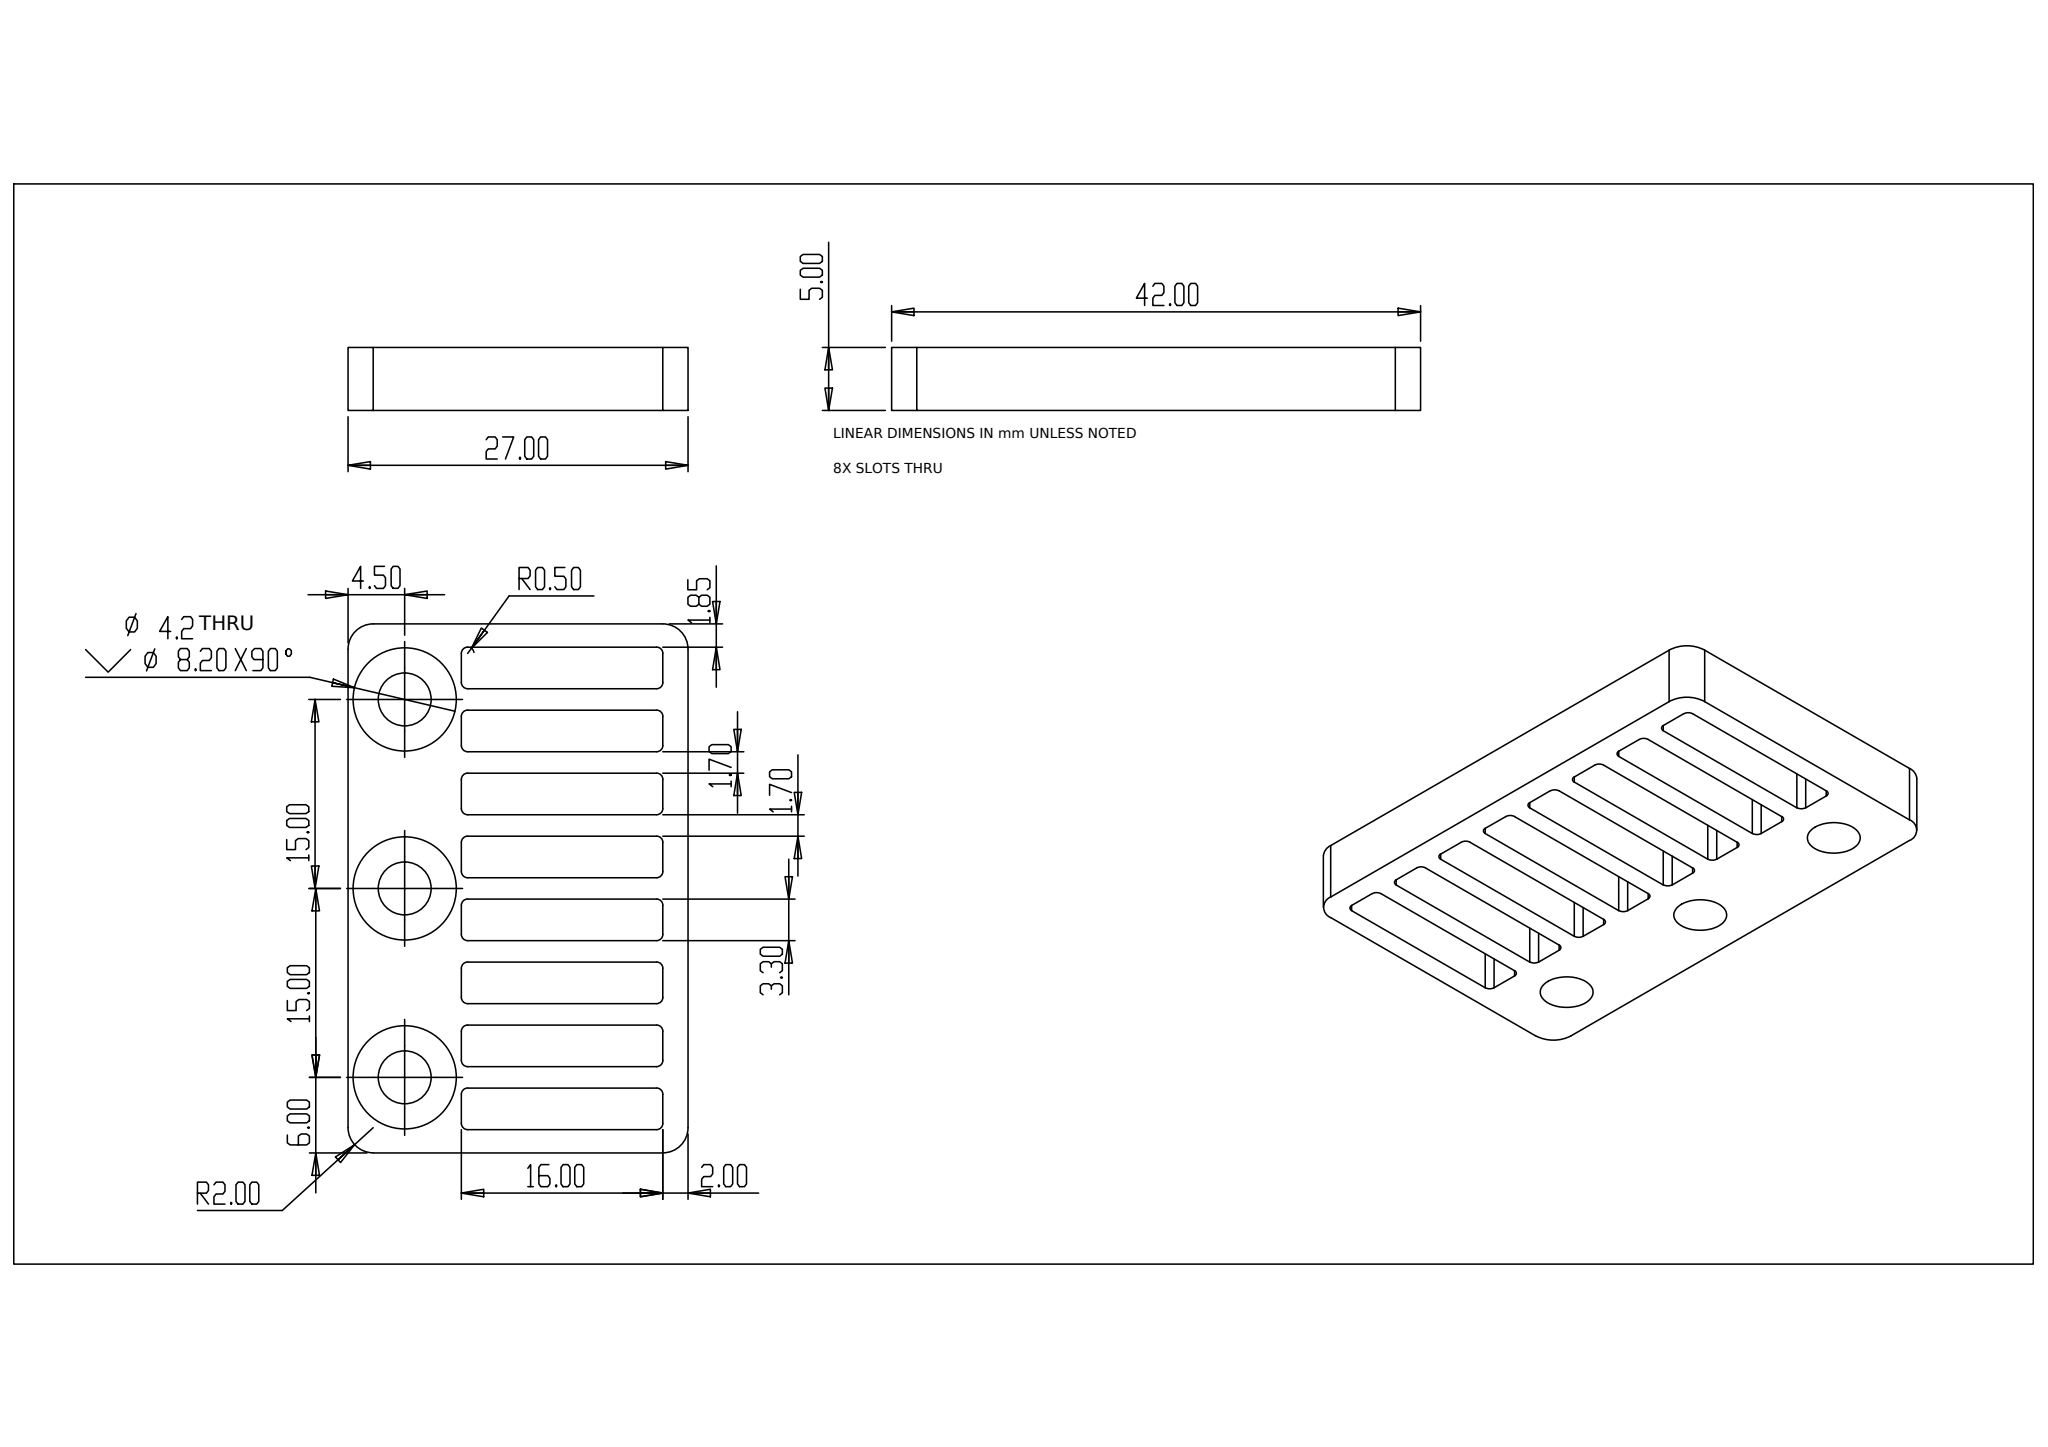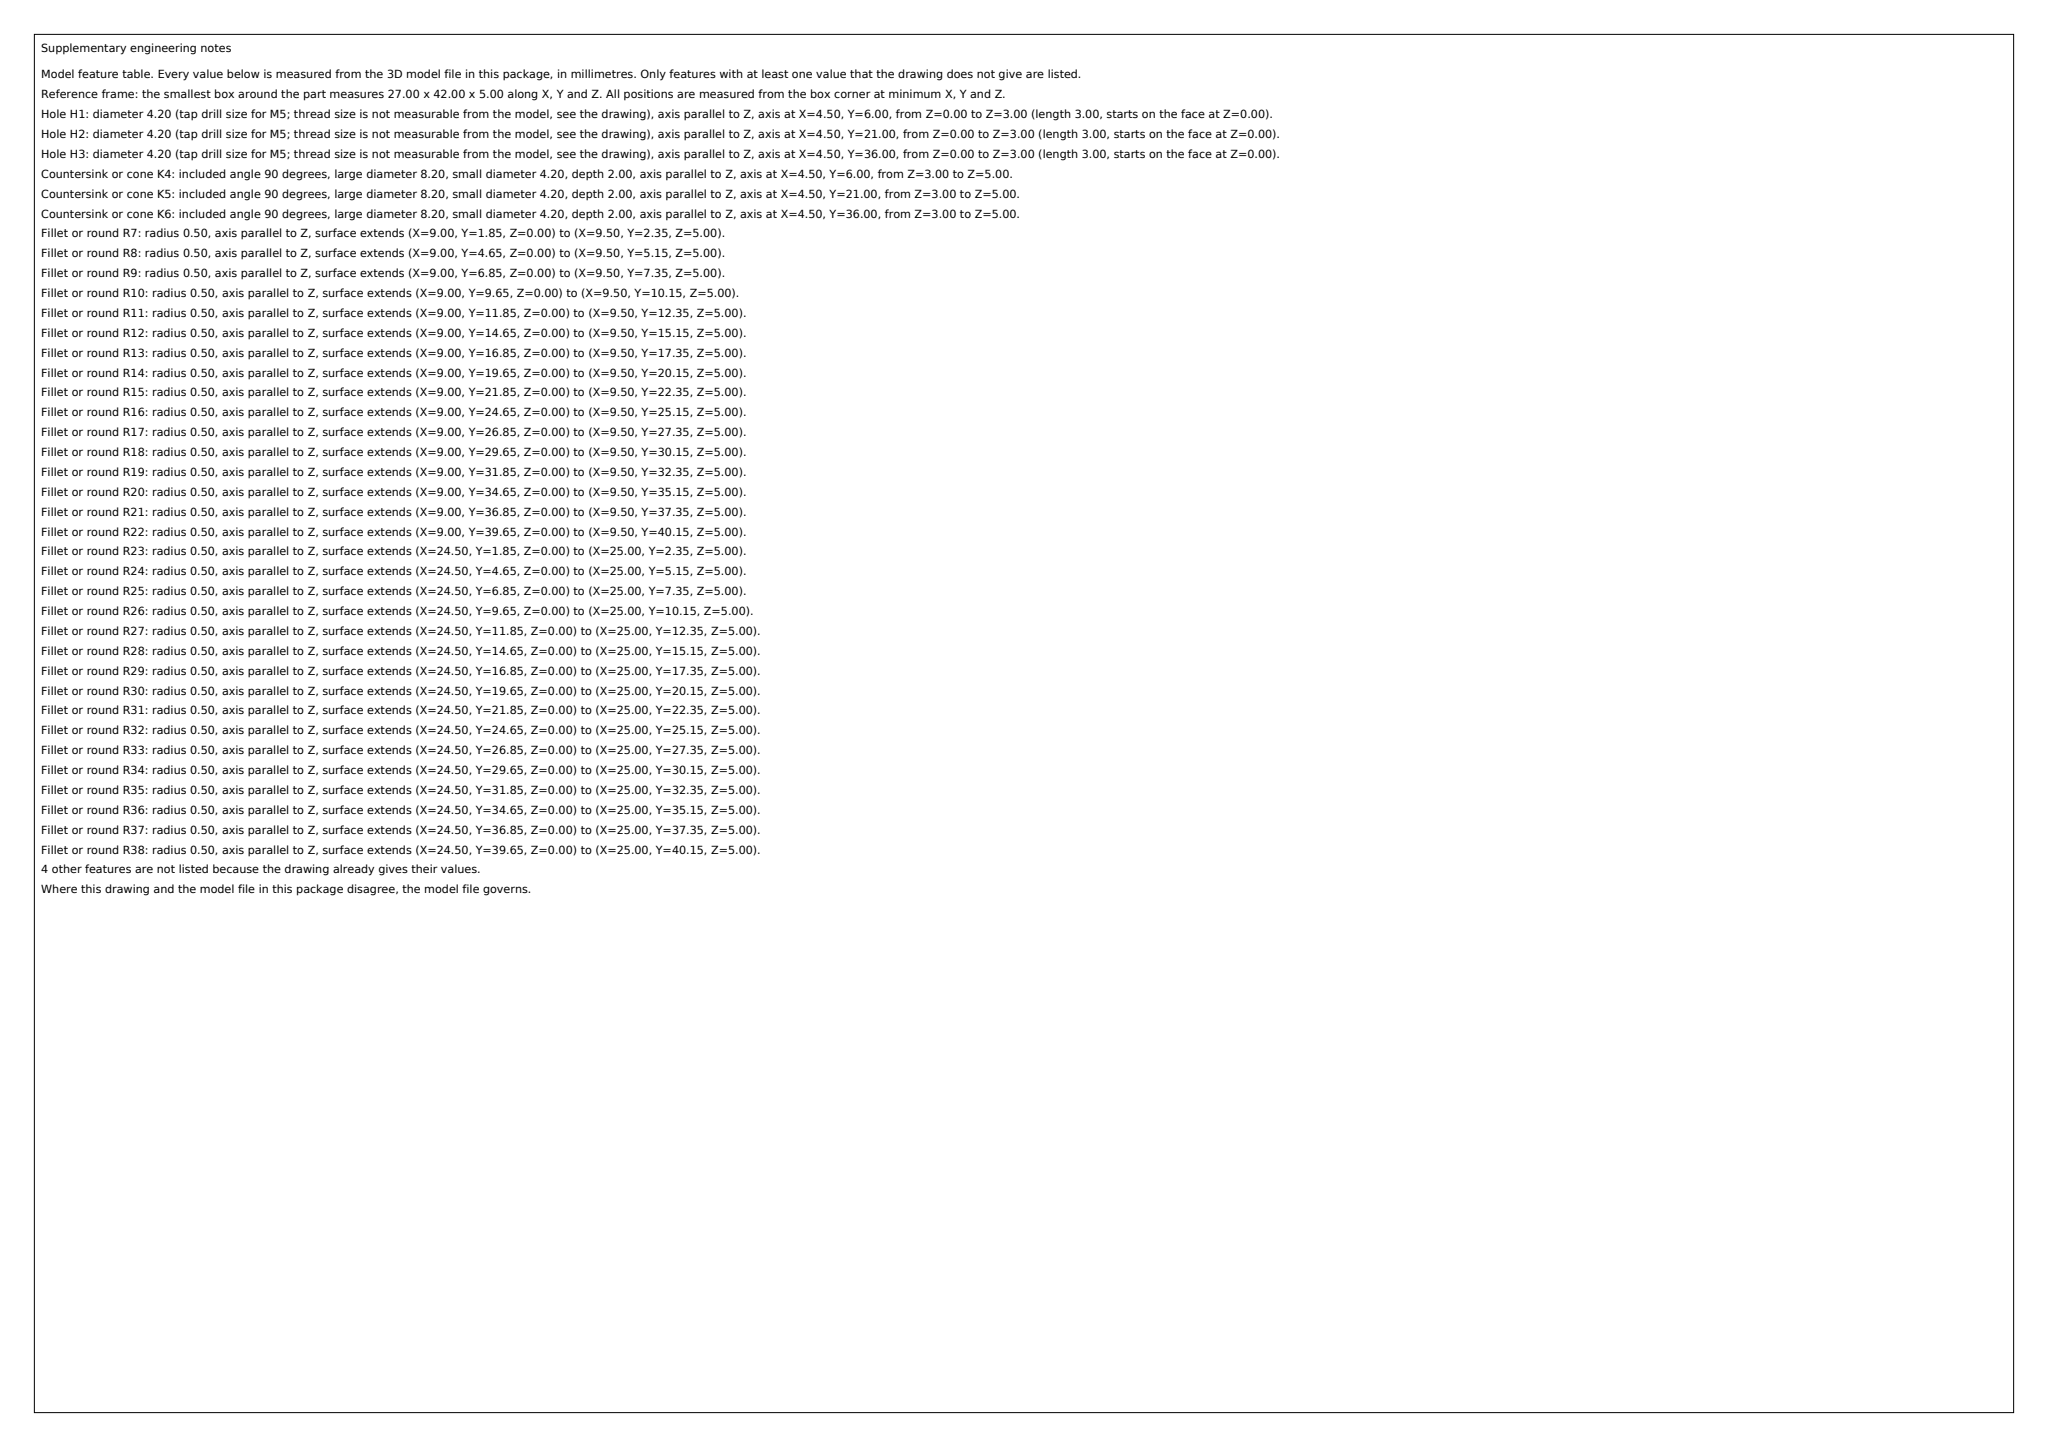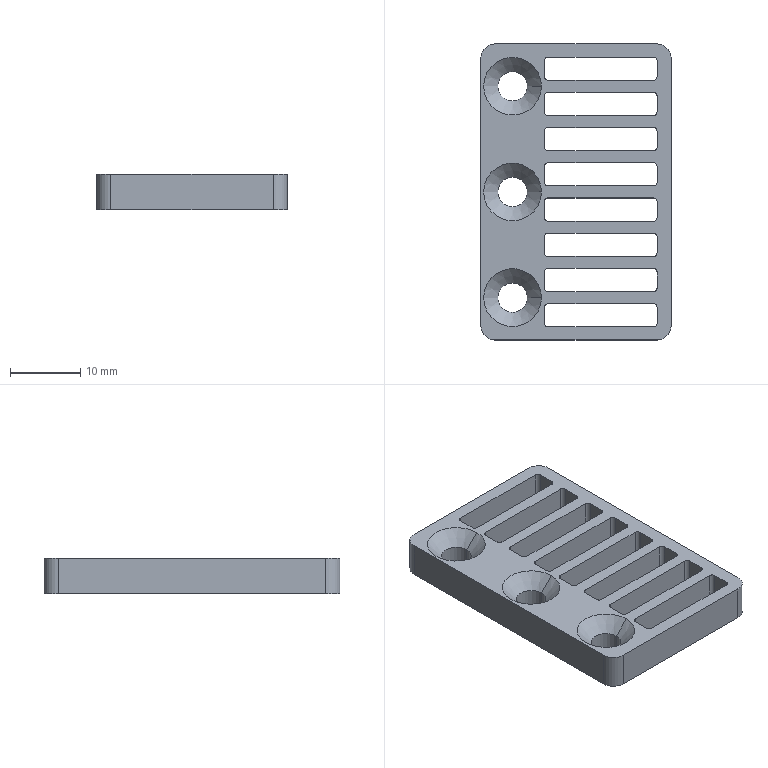Part | SolidWorks | mm | 1 solid | 86 faces | box 27 x 42 x 5 mm | volume 3237 mm3 | cylinder 42 | plane 38 | cone 6 | commonest cylinder face diameters 1 x32 4.2 x6 4 x4
build123d program:
from build123d import *

# Parameters (mm, degrees)
BOSS_EXTRUDE1_DEPTH = 5
CHAMFER1_SIZE       = 2


with BuildPart() as part:
    # Sketch1 → Boss-Extrude1 (new body)
    with BuildSketch(Plane.XY):
        with BuildLine():
            Line((-11.5, -21), (11.5, -21))
            ThreePointArc((11.5, -21), (12.914, -20.414), (13.5, -19))
            Line((13.5, -19), (13.5, 19))
            ThreePointArc((13.5, 19), (12.914, 20.414), (11.5, 21))
            Line((11.5, 21), (-11.5, 21))
            ThreePointArc((-11.5, 21), (-12.914, 20.414), (-13.5, 19))
            Line((-13.5, 19), (-13.5, -19))
            ThreePointArc((-13.5, -19), (-12.914, -20.414), (-11.5, -21))
        make_face()
        with BuildLine():
            Line((-4.5, -11.35), (-4.5, -13.65))
            ThreePointArc((-4.5, -13.65), (-4.354, -14.004), (-4, -14.15))
            Line((-4, -14.15), (11, -14.15))
            ThreePointArc((11, -14.15), (11.354, -14.004), (11.5, -13.65))
            Line((11.5, -13.65), (11.5, -11.35))
            ThreePointArc((11.5, -11.35), (11.354, -10.996), (11, -10.85))
            Line((11, -10.85), (-4, -10.85))
            ThreePointArc((-4, -10.85), (-4.354, -10.996), (-4.5, -11.35))
        make_face(mode=Mode.SUBTRACT)
        with BuildLine():
            Line((-4.5, 3.65), (-4.5, 1.35))
            ThreePointArc((-4.5, 1.35), (-4.354, 0.9964), (-4, 0.85))
            Line((-4, 0.85), (11, 0.85))
            ThreePointArc((11, 0.85), (11.354, 0.9964), (11.5, 1.35))
            Line((11.5, 1.35), (11.5, 3.65))
            ThreePointArc((11.5, 3.65), (11.354, 4.004), (11, 4.15))
            Line((11, 4.15), (-4, 4.15))
            ThreePointArc((-4, 4.15), (-4.354, 4.004), (-4.5, 3.65))
        make_face(mode=Mode.SUBTRACT)
        with BuildLine():
            Line((-4.5, 18.65), (-4.5, 16.35))
            ThreePointArc((-4.5, 16.35), (-4.354, 15.996), (-4, 15.85))
            Line((-4, 15.85), (11, 15.85))
            ThreePointArc((11, 15.85), (11.354, 15.996), (11.5, 16.35))
            Line((11.5, 16.35), (11.5, 18.65))
            ThreePointArc((11.5, 18.65), (11.354, 19.004), (11, 19.15))
            Line((11, 19.15), (-4, 19.15))
            ThreePointArc((-4, 19.15), (-4.354, 19.004), (-4.5, 18.65))
        make_face(mode=Mode.SUBTRACT)
        with BuildLine():
            Line((-4.5, -1.35), (-4.5, -3.65))
            ThreePointArc((-4.5, -3.65), (-4.354, -4.004), (-4, -4.15))
            Line((-4, -4.15), (11, -4.15))
            ThreePointArc((11, -4.15), (11.354, -4.004), (11.5, -3.65))
            Line((11.5, -3.65), (11.5, -1.35))
            ThreePointArc((11.5, -1.35), (11.354, -0.9964), (11, -0.85))
            Line((11, -0.85), (-4, -0.85))
            ThreePointArc((-4, -0.85), (-4.354, -0.9964), (-4.5, -1.35))
        make_face(mode=Mode.SUBTRACT)
        with BuildLine():
            Line((-4.5, 13.65), (-4.5, 11.35))
            ThreePointArc((-4.5, 11.35), (-4.354, 10.996), (-4, 10.85))
            Line((-4, 10.85), (11, 10.85))
            ThreePointArc((11, 10.85), (11.354, 10.996), (11.5, 11.35))
            Line((11.5, 11.35), (11.5, 13.65))
            ThreePointArc((11.5, 13.65), (11.354, 14.004), (11, 14.15))
            Line((11, 14.15), (-4, 14.15))
            ThreePointArc((-4, 14.15), (-4.354, 14.004), (-4.5, 13.65))
        make_face(mode=Mode.SUBTRACT)
        with BuildLine():
            Line((-4.5, -16.35), (-4.5, -18.65))
            ThreePointArc((-4.5, -18.65), (-4.354, -19.004), (-4, -19.15))
            Line((-4, -19.15), (11, -19.15))
            ThreePointArc((11, -19.15), (11.354, -19.004), (11.5, -18.65))
            Line((11.5, -18.65), (11.5, -16.35))
            ThreePointArc((11.5, -16.35), (11.354, -15.996), (11, -15.85))
            Line((11, -15.85), (-4, -15.85))
            ThreePointArc((-4, -15.85), (-4.354, -15.996), (-4.5, -16.35))
        make_face(mode=Mode.SUBTRACT)
        with BuildLine():
            Line((-4.5, -6.35), (-4.5, -8.65))
            ThreePointArc((-4.5, -8.65), (-4.354, -9.004), (-4, -9.15))
            Line((-4, -9.15), (11, -9.15))
            ThreePointArc((11, -9.15), (11.354, -9.004), (11.5, -8.65))
            Line((11.5, -8.65), (11.5, -6.35))
            ThreePointArc((11.5, -6.35), (11.354, -5.996), (11, -5.85))
            Line((11, -5.85), (-4, -5.85))
            ThreePointArc((-4, -5.85), (-4.354, -5.996), (-4.5, -6.35))
        make_face(mode=Mode.SUBTRACT)
        with BuildLine():
            Line((-4.5, 8.65), (-4.5, 6.35))
            ThreePointArc((-4.5, 6.35), (-4.354, 5.996), (-4, 5.85))
            Line((-4, 5.85), (11, 5.85))
            ThreePointArc((11, 5.85), (11.354, 5.996), (11.5, 6.35))
            Line((11.5, 6.35), (11.5, 8.65))
            ThreePointArc((11.5, 8.65), (11.354, 9.004), (11, 9.15))
            Line((11, 9.15), (-4, 9.15))
            ThreePointArc((-4, 9.15), (-4.354, 9.004), (-4.5, 8.65))
        make_face(mode=Mode.SUBTRACT)
        with BuildLine():
            ThreePointArc((-11.1, -15), (-9, -17.1), (-6.9, -15))
            ThreePointArc((-6.9, -15), (-9, -12.9), (-11.1, -15))
        make_face(mode=Mode.SUBTRACT)
        with BuildLine():
            ThreePointArc((-9, -2.1), (-6.9, 0), (-9, 2.1))
            ThreePointArc((-9, 2.1), (-11.1, 0), (-9, -2.1))
        make_face(mode=Mode.SUBTRACT)
        with BuildLine():
            ThreePointArc((-11.1, 15), (-9, 12.9), (-6.9, 15))
            ThreePointArc((-6.9, 15), (-9, 17.1), (-11.1, 15))
        make_face(mode=Mode.SUBTRACT)
    extrude(amount=BOSS_EXTRUDE1_DEPTH)

    # Chamfer1
    chamfer1_edges = [part.edges().sort_by_distance(p)[0] for p in [
        (-11.1, 15, 5),
        (-11.1, -15, 5),
        (-9, -2.1, 5),
    ]]
    chamfer(chamfer1_edges, length=CHAMFER1_SIZE)


solid = part.part